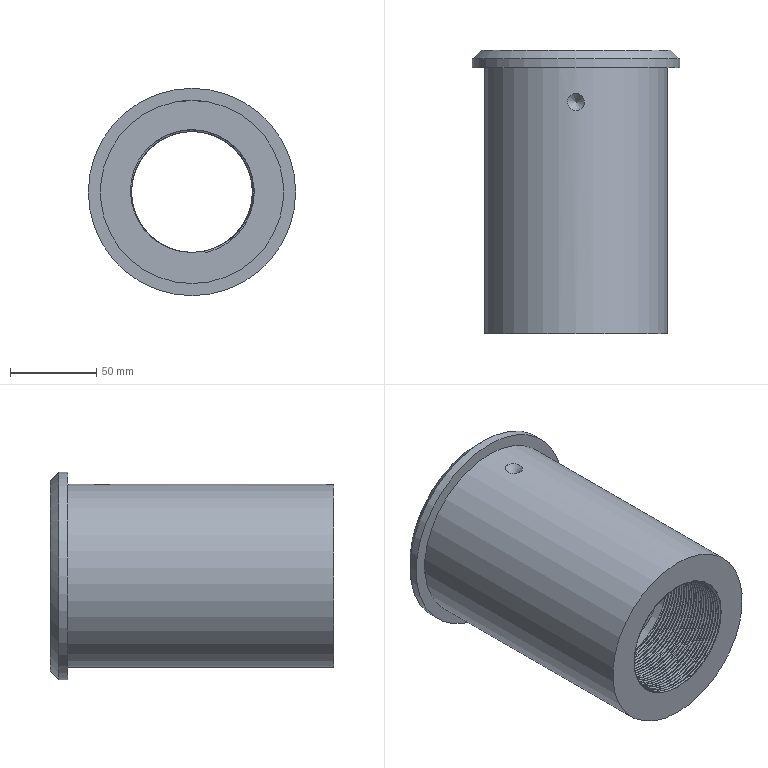Component | NX | BUSHING | 1 solid | 17 faces | volume 795450 mm3 | cylinder 8 | plane 5 | cone 2 | spline 2 | commonest cylinder face diameters 72 x2 10 x2 120 x1 106 x1 70 x1 80 x1